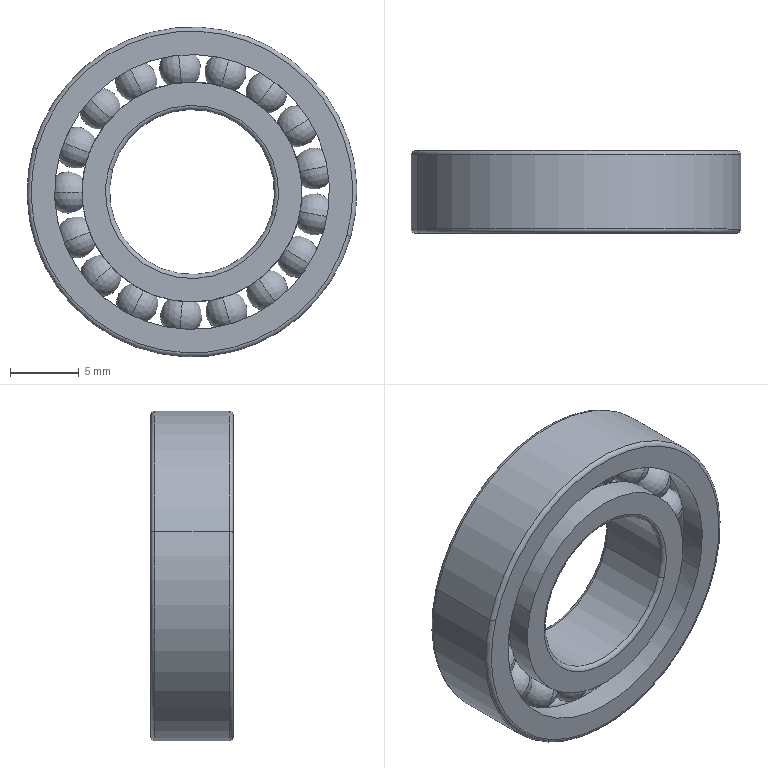Component | SolidWorks | deep groove ball bearings gb-1 | 1 solid | 112 faces | volume 1508 mm3 | torus 62 | sphere 34 | cylinder 12 | plane 4 | commonest cylinder face diameters 20 x4 16 x4 24 x2 12 x2